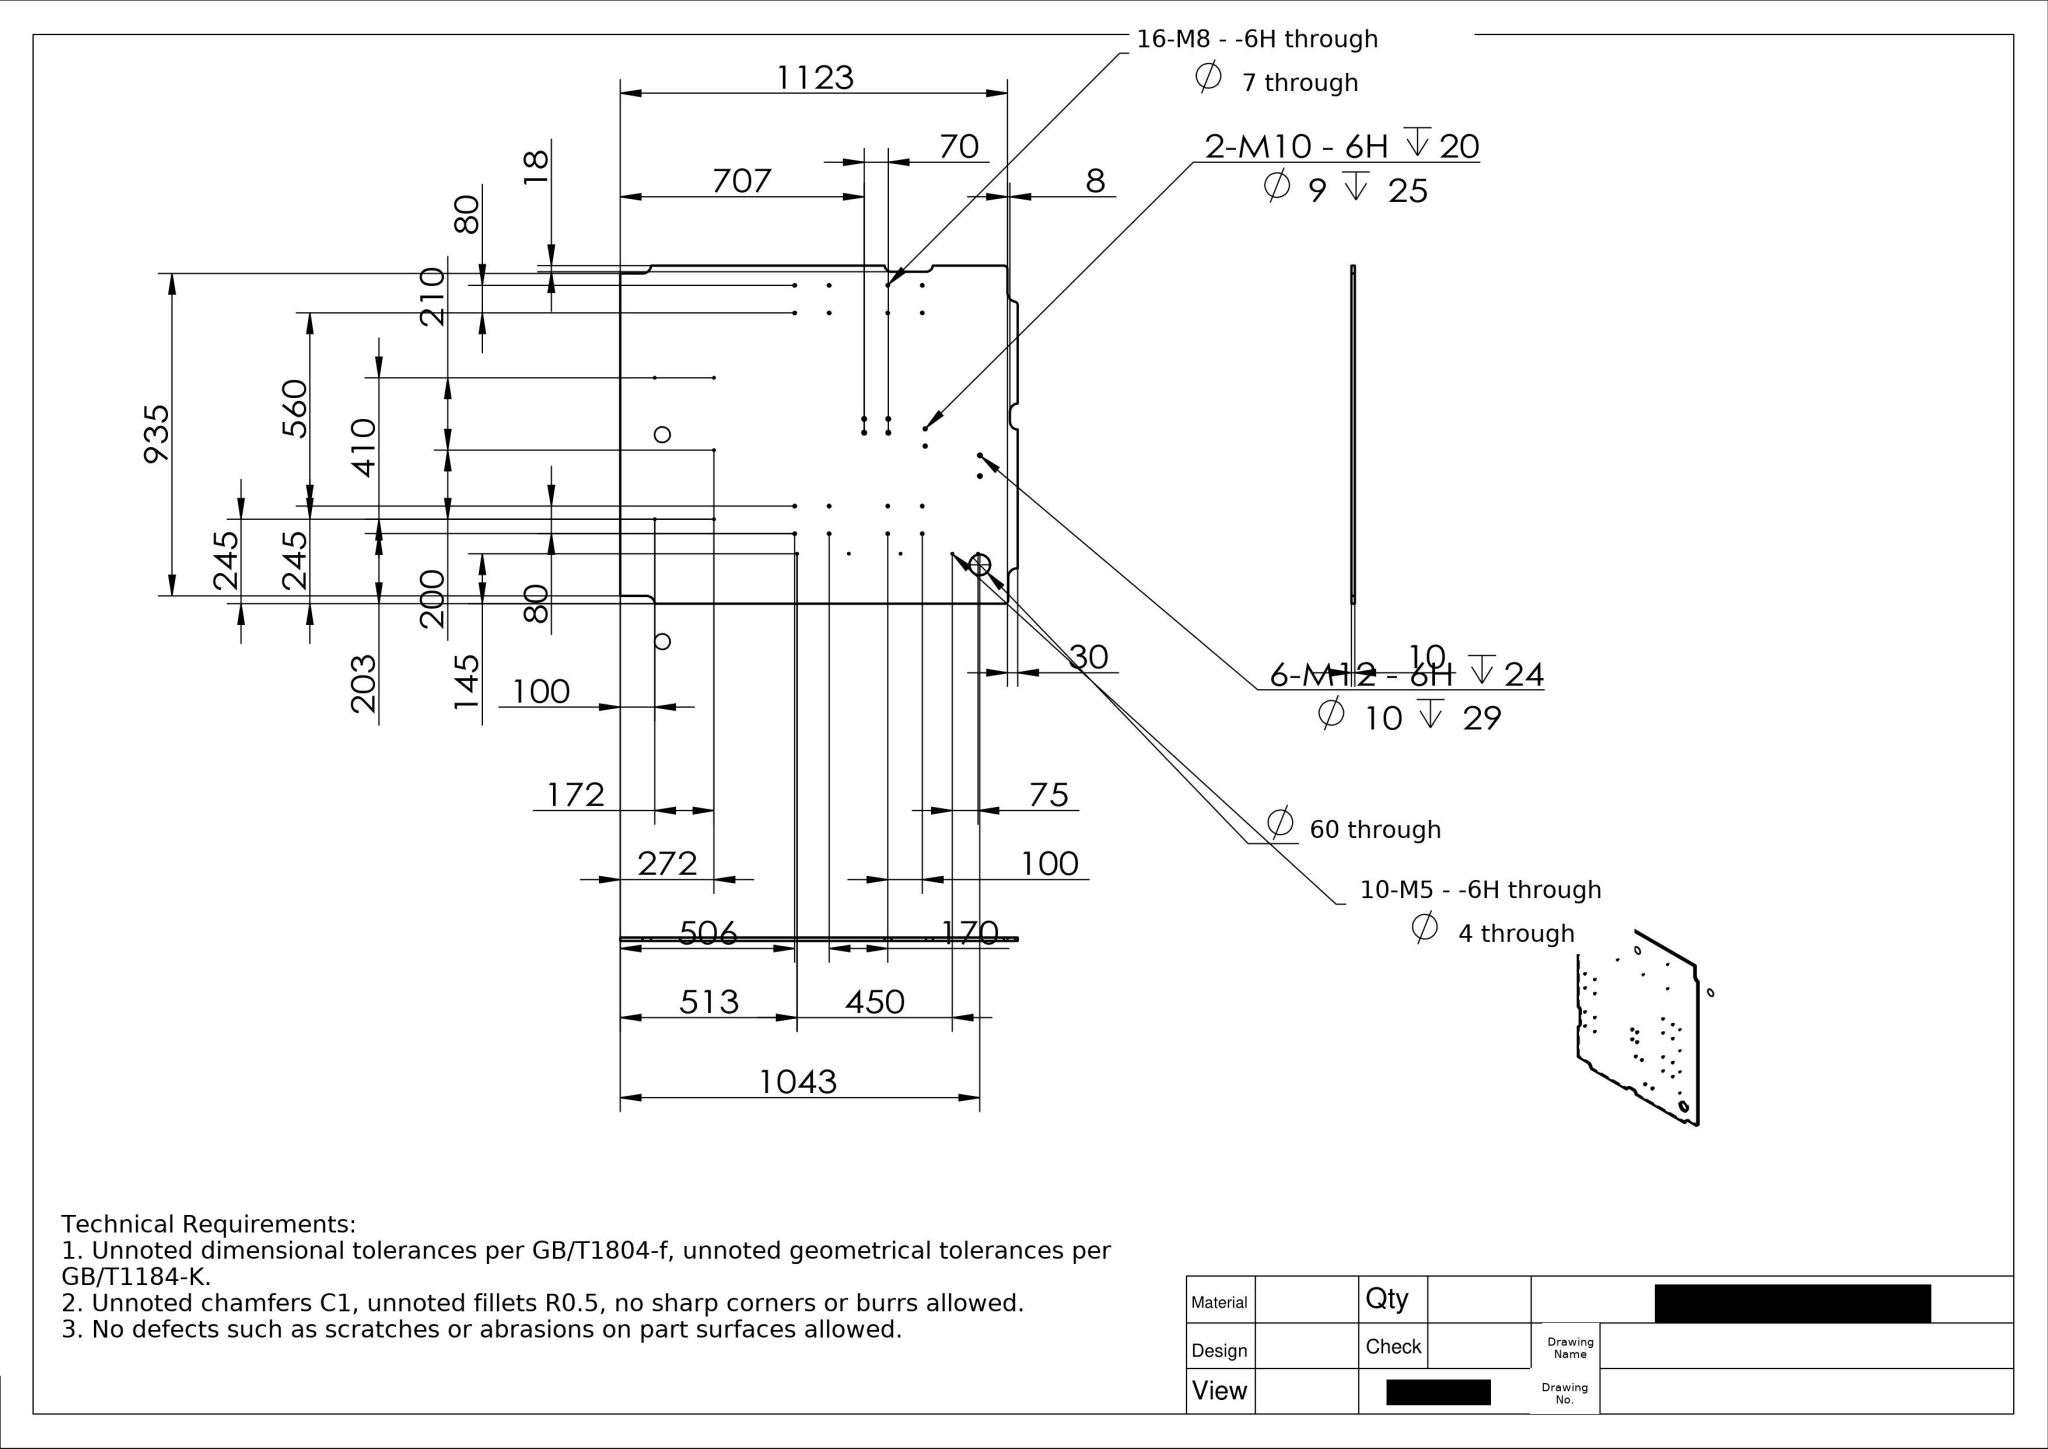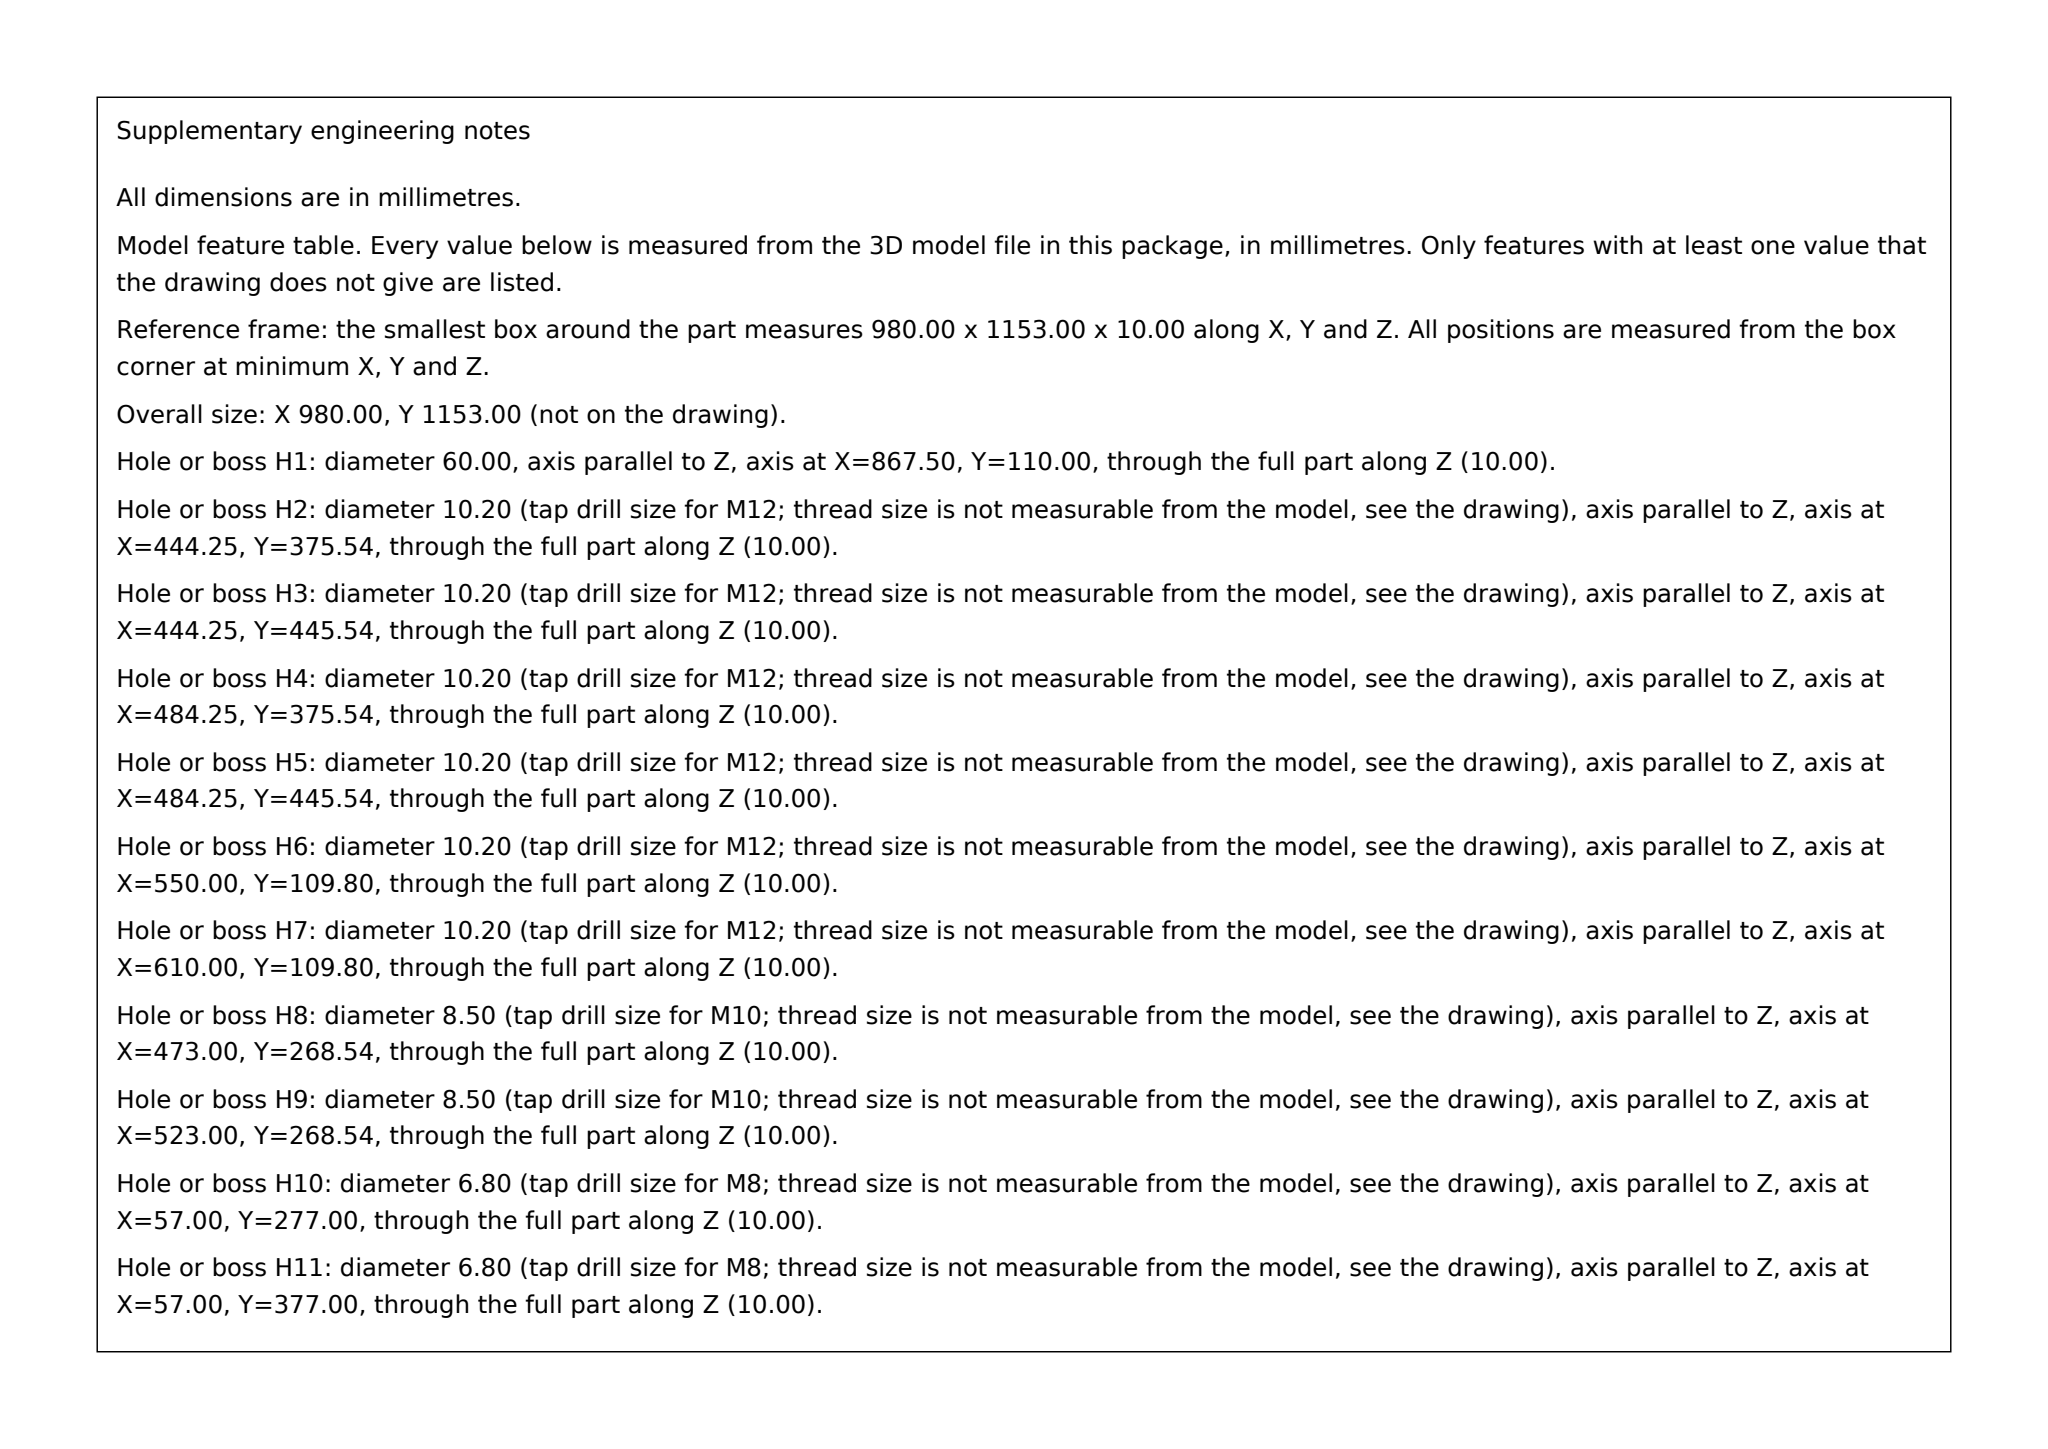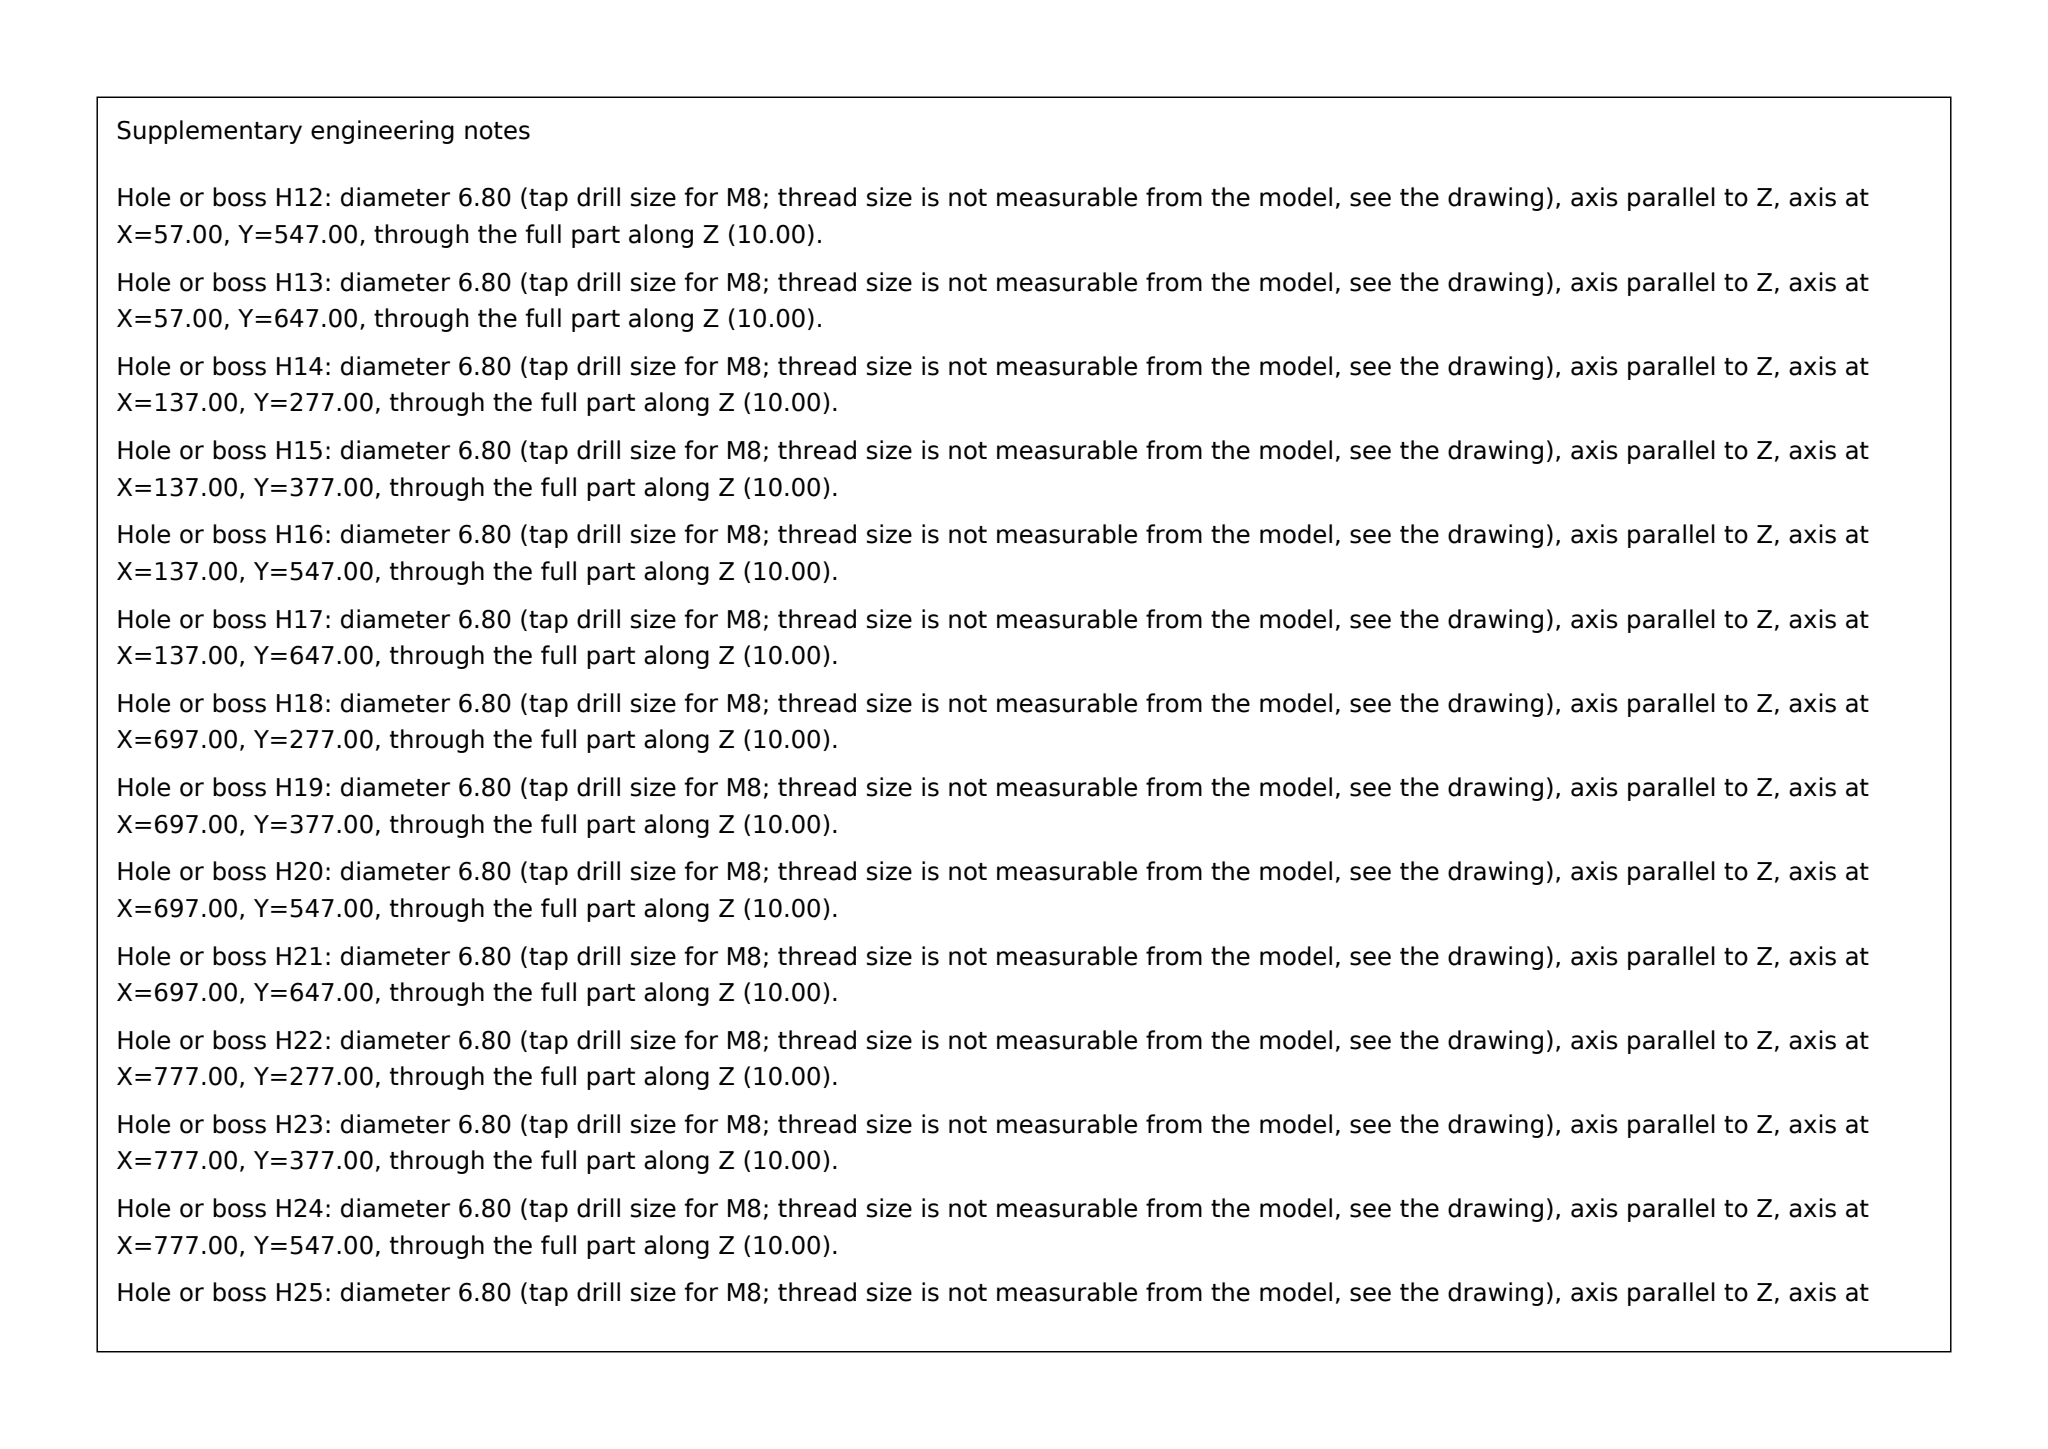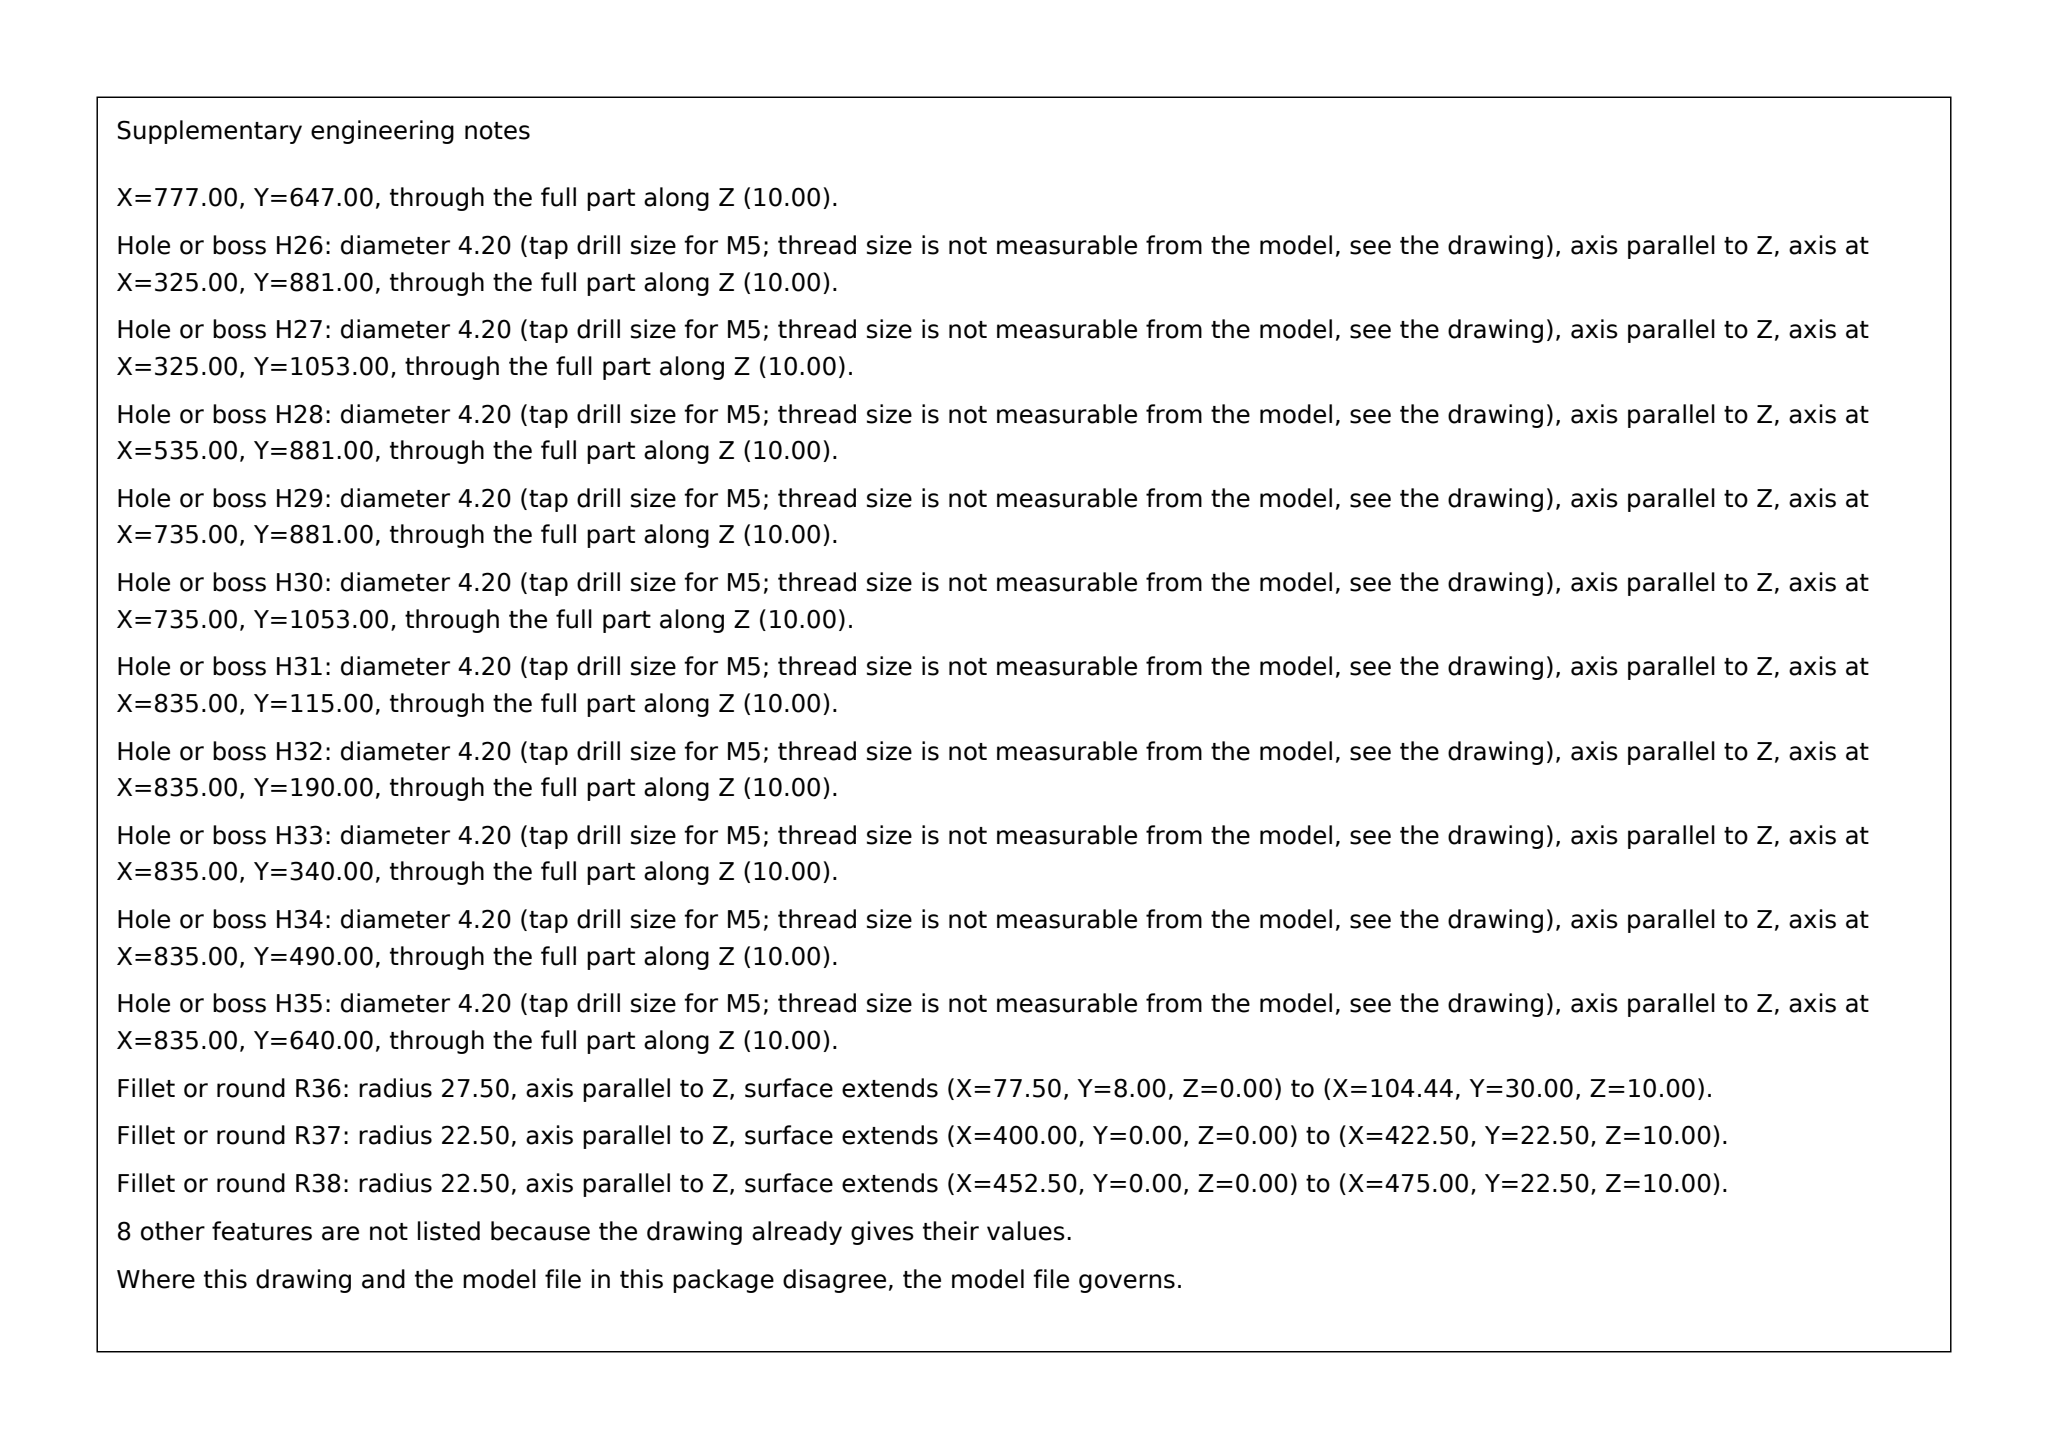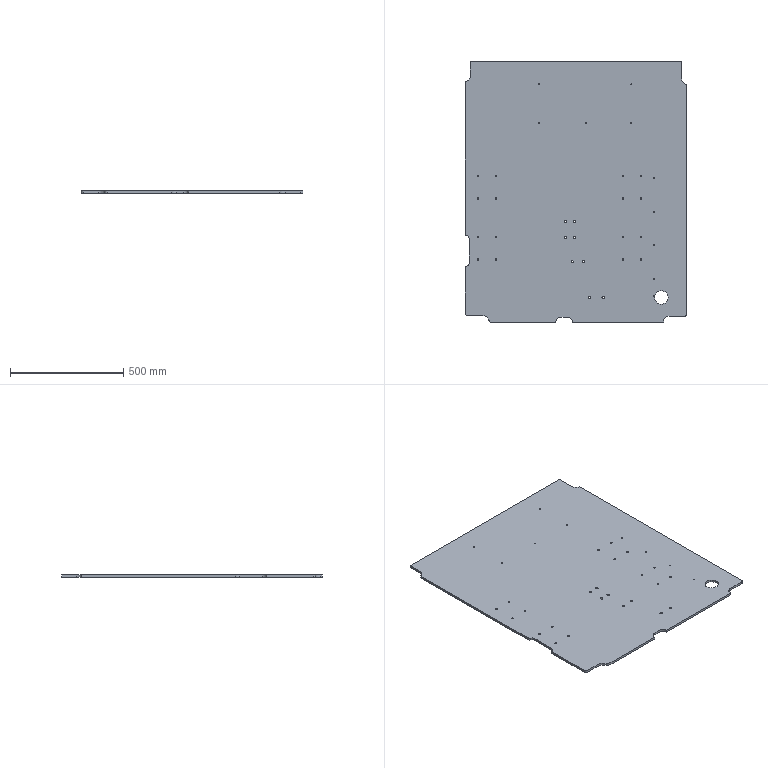Part | SolidWorks | mm | 1 solid | 95 faces | box 980 x 1153 x 10 mm | volume 11122889 mm3 | cylinder 81 | plane 14 | commonest cylinder face diameters 6.8 x32 4.2 x20 10.2 x12 8.5 x4 50 x3 20 x3 60 x2 40 x2
build123d program:
from build123d import *

# Parameters (mm, degrees)
SKETCH1_W              = 1030
SKETCH1_H              = 1153
BOSS_EXTRUDE1_DEPTH    = 10
FILLET1_R              = 10
M5_TAPPED_HOLE1_D      = 4.2
SKETCH46_W             = 118.194
SKETCH46_H             = 1894.415
CUT_EXTRUDE13_DEPTH    = 1547.095
M12_TAPPED_HOLE1_D     = 10.2
M12_TAPPED_HOLE1_DEPTH = 29.25
M12_TAPPED_HOLE1_TIP   = 3.064
M10_TAPPED_HOLE3_D     = 8.5
M10_TAPPED_HOLE3_DEPTH = 24.5
M10_TAPPED_HOLE3_TIP   = 2.554
M12_TAPPED_HOLE2_D     = 10.2
M12_TAPPED_HOLE2_DEPTH = 29.25
M12_TAPPED_HOLE2_TIP   = 3.064
M8_TAPPED_HOLE1_D      = 6.8
SKETCH55_R             = 30
CUT_EXTRUDE14_DEPTH    = 1530.554
CUT_EXTRUDE16_DEPTH    = 10
FILLET2_R              = 10


with BuildPart() as part:
    # Sketch1 → Boss-Extrude1 (new body)
    with BuildSketch(Plane.XY):
        with Locations((515, 576.5)):
            Rectangle(SKETCH1_W, SKETCH1_H)
    extrude(amount=BOSS_EXTRUDE1_DEPTH)

    # Fillet1
    fillet1_edges = [part.edges().sort_by_distance(p)[0] for p in [
        (1030, 0, 5),
        (0, 0, 5),
    ]]
    fillet(fillet1_edges, radius=FILLET1_R)

    # M5 Tapped Hole1 (through all)
    with Locations(Plane.XY.offset(10)):
        with Locations((560, 881), (860, 190), (860, 340), (860, 490), (350, 1053), (350, 881), (760, 1053), (760, 881), (860, 640), (860, 115)):
            Hole(M5_TAPPED_HOLE1_D / 2)

    # Sketch46 → Cut-Extrude13 (cut, through all)
    with BuildSketch(Plane.XY.offset(10)):
        with Locations((-34.097, 851.22)):
            Rectangle(SKETCH46_W, SKETCH46_H)
    cut_extrude13 = extrude(amount=-CUT_EXTRUDE13_DEPTH, mode=Mode.SUBTRACT)

    # Mirror1: Cut-Extrude13 across plane
    add(cut_extrude13.mirror(Plane(origin=(515, 0, 0), x_dir=(0, 0, 1), z_dir=(1, 0, 0))), mode=Mode.SUBTRACT)

    # M12 Tapped Hole1
    with Locations(Plane.XY.offset(10)):
        with Locations((469.25, 445.542), (469.25, 375.542), (509.25, 375.542), (509.25, 445.542)):
            Hole(M12_TAPPED_HOLE1_D / 2, depth=M12_TAPPED_HOLE1_DEPTH)
            with Locations((0, 0, -(M12_TAPPED_HOLE1_DEPTH + M12_TAPPED_HOLE1_TIP / 2))):  # 118° drill point
                Cone(0, M12_TAPPED_HOLE1_D / 2, M12_TAPPED_HOLE1_TIP, mode=Mode.SUBTRACT)

    # M10 Tapped Hole3
    with Locations(Plane.XY.offset(10)):
        with Locations((498, 268.542), (548, 268.542)):
            Hole(M10_TAPPED_HOLE3_D / 2, depth=M10_TAPPED_HOLE3_DEPTH)
            with Locations((0, 0, -(M10_TAPPED_HOLE3_DEPTH + M10_TAPPED_HOLE3_TIP / 2))):  # 118° drill point
                Cone(0, M10_TAPPED_HOLE3_D / 2, M10_TAPPED_HOLE3_TIP, mode=Mode.SUBTRACT)

    # M12 Tapped Hole2
    with Locations(Plane.XY.offset(10)):
        with Locations((575, 109.8), (635, 109.8)):
            Hole(M12_TAPPED_HOLE2_D / 2, depth=M12_TAPPED_HOLE2_DEPTH)
            with Locations((0, 0, -(M12_TAPPED_HOLE2_DEPTH + M12_TAPPED_HOLE2_TIP / 2))):  # 118° drill point
                Cone(0, M12_TAPPED_HOLE2_D / 2, M12_TAPPED_HOLE2_TIP, mode=Mode.SUBTRACT)

    # M8 Tapped Hole1 (through all)
    with Locations(Plane.XY.offset(10)):
        with Locations((722, 277), (722, 377), (802, 377), (802, 277), (82, 277), (82, 377), (162, 277), (162, 377), (162, 547), (82, 547), (82, 647), (162, 647), (722, 547), (722, 647), (802, 647), (802, 547)):
            Hole(M8_TAPPED_HOLE1_D / 2)

    # Sketch55 → Cut-Extrude14 (cut, through all)
    with BuildSketch(Plane.XY.offset(10)):
        with Locations((892.5, 110)):
            Circle(SKETCH55_R)
        with BuildLine():
            Line((42.5, 366), (42.5, 266))
            ThreePointArc((42.5, 266), (22.5, 246), (2.5, 266))
            Line((2.5, 266), (2.5, 366))
            ThreePointArc((2.5, 366), (22.5, 386), (42.5, 366))
        make_face()
        with BuildLine():
            Line((102.5, -25), (-29.53, -25))
            ThreePointArc((-29.53, -25), (-57.03, 2.5), (-29.53, 30))
            Line((-29.53, 30), (102.5, 30))
            ThreePointArc((102.5, 30), (130, 2.5), (102.5, -25))
        make_face()
        with BuildLine():
            Line((477.5, -22.5), (447.5, -22.5))
            ThreePointArc((447.5, -22.5), (425, 0), (447.5, 22.5))
            Line((447.5, 22.5), (477.5, 22.5))
            ThreePointArc((477.5, 22.5), (500, 0), (477.5, -22.5))
        make_face()
        with BuildLine():
            Line((927.5, 27.5), (1025.664, 27.5))
            ThreePointArc((1025.664, 27.5), (1050.664, 2.5), (1025.664, -22.5))
            Line((1025.664, -22.5), (927.5, -22.5))
            ThreePointArc((927.5, -22.5), (902.5, 2.5), (927.5, 27.5))
        make_face()
    extrude(amount=-CUT_EXTRUDE14_DEPTH, mode=Mode.SUBTRACT)

    # Sketch57 → Cut-Extrude16 (cut)
    with BuildSketch(Plane(origin=(0, 0, 0), x_dir=(-1, 0, 0), z_dir=(0, 0, -1))):
        with BuildLine():
            Line((-47.5, 1088.419), (-47.5, 1182.734))
            ThreePointArc((-47.5, 1182.734), (-22.5, 1207.734), (2.5, 1182.734))
            Line((2.5, 1182.734), (2.5, 1088.419))
            ThreePointArc((2.5, 1088.419), (-22.5, 1063.419), (-47.5, 1088.419))
        make_face()
        with BuildLine():
            Line((-1032.5, 1077), (-1032.5, 1177.523))
            ThreePointArc((-1032.5, 1177.523), (-1007.5, 1202.523), (-982.5, 1177.523))
            Line((-982.5, 1177.523), (-982.5, 1077))
            ThreePointArc((-982.5, 1077), (-1007.5, 1052), (-1032.5, 1077))
        make_face()
    extrude(amount=-CUT_EXTRUDE16_DEPTH, mode=Mode.SUBTRACT)

    # Fillet2
    fillet2_edges = [part.edges().sort_by_distance(p)[0] for p in [
        (1005, 27.5, 5),
        (25, 30, 5),
        (129.886, 0, 5),
    ]]
    fillet(fillet2_edges, radius=FILLET2_R)


solid = part.part